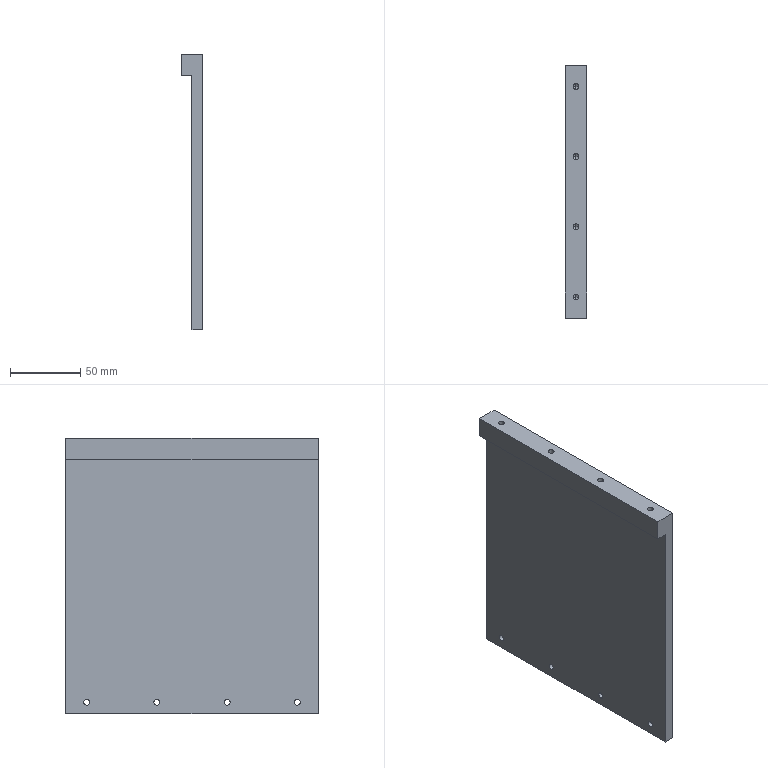Component | SolidWorks | P-SLJ-001-005-1 | 1 solid | 32 faces | box 15 x 180 x 196 mm | volume 283635 mm3 | cylinder 16 | cone 8 | plane 8 | commonest cylinder face diameters 4.2 x16 | material 45#
STEP:
#1=CARTESIAN_POINT('',(-14.213,3.346,40.769));
#2=VERTEX_POINT('',#1);
#3=CARTESIAN_POINT('',(-14.213,3.346,40.934));
#4=VERTEX_POINT('',#3);
#5=CARTESIAN_POINT('',(-14.213,3.346,40.852));
#6=DIRECTION('',(-1.,0.,0.));
#7=DIRECTION('',(0.,0.,1.));
#8=AXIS2_PLACEMENT_3D('',#5,#6,#7);
#9=CIRCLE('',#8,0.08268);
#10=EDGE_CURVE('',#2,#4,#9,.T.);
#11=ORIENTED_EDGE('',*,*,#10,.F.);
#12=CARTESIAN_POINT('',(-14.508,3.346,40.769));
#13=VERTEX_POINT('',#12);
#14=CARTESIAN_POINT('',(-14.508,3.346,40.769));
#15=DIRECTION('',(-1.,0.,0.));
#16=VECTOR('',#15,39.37);
#17=LINE('',#14,#16);
#18=EDGE_CURVE('',#2,#13,#17,.T.);
#19=ORIENTED_EDGE('',*,*,#18,.T.);
#20=CARTESIAN_POINT('',(-14.508,3.346,40.934));
#21=VERTEX_POINT('',#20);
#22=CARTESIAN_POINT('',(-14.508,3.346,40.852));
#23=DIRECTION('',(-1.,0.,0.));
#24=DIRECTION('',(0.,0.,1.));
#25=AXIS2_PLACEMENT_3D('',#22,#23,#24);
#26=CIRCLE('',#25,0.08268);
#27=EDGE_CURVE('',#13,#21,#26,.T.);
#28=ORIENTED_EDGE('',*,*,#27,.T.);
#29=CARTESIAN_POINT('',(-14.508,3.346,40.934));
#30=DIRECTION('',(-1.,0.,0.));
#31=VECTOR('',#30,39.37);
#32=LINE('',#29,#31);
#33=EDGE_CURVE('',#4,#21,#32,.T.);
#34=ORIENTED_EDGE('',*,*,#33,.F.);
#35=EDGE_LOOP('',(#11,#19,#28,#34));
#36=FACE_OUTER_BOUND('',#35,.T.);
#37=CARTESIAN_POINT('',(-14.508,3.346,40.852));
#38=DIRECTION('',(-1.,0.,0.));
#39=DIRECTION('',(0.,0.,1.));
#40=AXIS2_PLACEMENT_3D('',#37,#38,#39);
#41=CYLINDRICAL_SURFACE('',#40,0.08268);
#42=ADVANCED_FACE('',(#36),#41,.F.);
#43=CARTESIAN_POINT('',(-14.213,1.378,40.769));
#44=VERTEX_POINT('',#43);
#45=CARTESIAN_POINT('',(-14.213,1.378,40.934));
#46=VERTEX_POINT('',#45);
#47=CARTESIAN_POINT('',(-14.213,1.378,40.852));
#48=DIRECTION('',(-1.,0.,0.));
#49=DIRECTION('',(0.,0.,1.));
#50=AXIS2_PLACEMENT_3D('',#47,#48,#49);
#51=CIRCLE('',#50,0.08268);
#52=EDGE_CURVE('',#44,#46,#51,.T.);
#53=ORIENTED_EDGE('',*,*,#52,.F.);
#54=CARTESIAN_POINT('',(-14.508,1.378,40.769));
#55=VERTEX_POINT('',#54);
#56=CARTESIAN_POINT('',(-14.508,1.378,40.769));
#57=DIRECTION('',(-1.,0.,0.));
#58=VECTOR('',#57,39.37);
#59=LINE('',#56,#58);
#60=EDGE_CURVE('',#44,#55,#59,.T.);
#61=ORIENTED_EDGE('',*,*,#60,.T.);
#62=CARTESIAN_POINT('',(-14.508,1.378,40.934));
#63=VERTEX_POINT('',#62);
#64=CARTESIAN_POINT('',(-14.508,1.378,40.852));
#65=DIRECTION('',(-1.,0.,0.));
#66=DIRECTION('',(0.,0.,1.));
#67=AXIS2_PLACEMENT_3D('',#64,#65,#66);
#68=CIRCLE('',#67,0.08268);
#69=EDGE_CURVE('',#55,#63,#68,.T.);
#70=ORIENTED_EDGE('',*,*,#69,.T.);
#71=CARTESIAN_POINT('',(-14.508,1.378,40.934));
#72=DIRECTION('',(-1.,0.,0.));
#73=VECTOR('',#72,39.37);
#74=LINE('',#71,#73);
#75=EDGE_CURVE('',#46,#63,#74,.T.);
#76=ORIENTED_EDGE('',*,*,#75,.F.);
#77=EDGE_LOOP('',(#53,#61,#70,#76));
#78=FACE_OUTER_BOUND('',#77,.T.);
#79=CARTESIAN_POINT('',(-14.508,1.378,40.852));
#80=DIRECTION('',(-1.,0.,0.));
#81=DIRECTION('',(0.,0.,1.));
#82=AXIS2_PLACEMENT_3D('',#79,#80,#81);
#83=CYLINDRICAL_SURFACE('',#82,0.08268);
#84=ADVANCED_FACE('',(#78),#83,.F.);
#85=CARTESIAN_POINT('',(-14.213,-0.5906,40.769));
#86=VERTEX_POINT('',#85);
#87=CARTESIAN_POINT('',(-14.213,-0.5906,40.934));
#88=VERTEX_POINT('',#87);
#89=CARTESIAN_POINT('',(-14.213,-0.5906,40.852));
#90=DIRECTION('',(-1.,0.,0.));
#91=DIRECTION('',(0.,0.,1.));
#92=AXIS2_PLACEMENT_3D('',#89,#90,#91);
#93=CIRCLE('',#92,0.08268);
#94=EDGE_CURVE('',#86,#88,#93,.T.);
#95=ORIENTED_EDGE('',*,*,#94,.F.);
#96=CARTESIAN_POINT('',(-14.508,-0.5906,40.769));
#97=VERTEX_POINT('',#96);
#98=CARTESIAN_POINT('',(-14.508,-0.5906,40.769));
#99=DIRECTION('',(-1.,0.,0.));
#100=VECTOR('',#99,39.37);
#101=LINE('',#98,#100);
#102=EDGE_CURVE('',#86,#97,#101,.T.);
#103=ORIENTED_EDGE('',*,*,#102,.T.);
#104=CARTESIAN_POINT('',(-14.508,-0.5906,40.934));
#105=VERTEX_POINT('',#104);
#106=CARTESIAN_POINT('',(-14.508,-0.5906,40.852));
#107=DIRECTION('',(-1.,0.,0.));
#108=DIRECTION('',(0.,0.,1.));
#109=AXIS2_PLACEMENT_3D('',#106,#107,#108);
#110=CIRCLE('',#109,0.08268);
#111=EDGE_CURVE('',#97,#105,#110,.T.);
#112=ORIENTED_EDGE('',*,*,#111,.T.);
#113=CARTESIAN_POINT('',(-14.508,-0.5906,40.934));
#114=DIRECTION('',(-1.,0.,0.));
#115=VECTOR('',#114,39.37);
#116=LINE('',#113,#115);
#117=EDGE_CURVE('',#88,#105,#116,.T.);
#118=ORIENTED_EDGE('',*,*,#117,.F.);
#119=EDGE_LOOP('',(#95,#103,#112,#118));
#120=FACE_OUTER_BOUND('',#119,.T.);
#121=CARTESIAN_POINT('',(-14.508,-0.5906,40.852));
#122=DIRECTION('',(-1.,0.,0.));
#123=DIRECTION('',(0.,0.,1.));
#124=AXIS2_PLACEMENT_3D('',#121,#122,#123);
#125=CYLINDRICAL_SURFACE('',#124,0.08268);
#126=ADVANCED_FACE('',(#120),#125,.F.);
#127=CARTESIAN_POINT('',(-14.213,-2.559,40.769));
#128=VERTEX_POINT('',#127);
#129=CARTESIAN_POINT('',(-14.213,-2.559,40.934));
#130=VERTEX_POINT('',#129);
#131=CARTESIAN_POINT('',(-14.213,-2.559,40.852));
#132=DIRECTION('',(-1.,0.,0.));
#133=DIRECTION('',(0.,0.,1.));
#134=AXIS2_PLACEMENT_3D('',#131,#132,#133);
#135=CIRCLE('',#134,0.08268);
#136=EDGE_CURVE('',#128,#130,#135,.T.);
#137=ORIENTED_EDGE('',*,*,#136,.F.);
#138=CARTESIAN_POINT('',(-14.508,-2.559,40.769));
#139=VERTEX_POINT('',#138);
#140=CARTESIAN_POINT('',(-14.508,-2.559,40.769));
#141=DIRECTION('',(-1.,0.,0.));
#142=VECTOR('',#141,39.37);
#143=LINE('',#140,#142);
#144=EDGE_CURVE('',#128,#139,#143,.T.);
#145=ORIENTED_EDGE('',*,*,#144,.T.);
#146=CARTESIAN_POINT('',(-14.508,-2.559,40.934));
#147=VERTEX_POINT('',#146);
#148=CARTESIAN_POINT('',(-14.508,-2.559,40.852));
#149=DIRECTION('',(-1.,0.,0.));
#150=DIRECTION('',(0.,0.,1.));
#151=AXIS2_PLACEMENT_3D('',#148,#149,#150);
#152=CIRCLE('',#151,0.08268);
#153=EDGE_CURVE('',#139,#147,#152,.T.);
#154=ORIENTED_EDGE('',*,*,#153,.T.);
#155=CARTESIAN_POINT('',(-14.508,-2.559,40.934));
#156=DIRECTION('',(-1.,0.,0.));
#157=VECTOR('',#156,39.37);
#158=LINE('',#155,#157);
#159=EDGE_CURVE('',#130,#147,#158,.T.);
#160=ORIENTED_EDGE('',*,*,#159,.F.);
#161=EDGE_LOOP('',(#137,#145,#154,#160));
#162=FACE_OUTER_BOUND('',#161,.T.);
#163=CARTESIAN_POINT('',(-14.508,-2.559,40.852));
#164=DIRECTION('',(-1.,0.,0.));
#165=DIRECTION('',(0.,0.,1.));
#166=AXIS2_PLACEMENT_3D('',#163,#164,#165);
#167=CYLINDRICAL_SURFACE('',#166,0.08268);
#168=ADVANCED_FACE('',(#162),#167,.F.);
#169=CARTESIAN_POINT('',(-14.591,3.346,47.702));
#170=VERTEX_POINT('',#169);
#171=CARTESIAN_POINT('',(-14.425,3.346,47.702));
#172=VERTEX_POINT('',#171);
#173=CARTESIAN_POINT('',(-14.508,3.346,47.702));
#174=DIRECTION('',(0.,0.,1.));
#175=DIRECTION('',(1.,0.,0.));
#176=AXIS2_PLACEMENT_3D('',#173,#174,#175);
#177=CIRCLE('',#176,0.08268);
#178=EDGE_CURVE('',#170,#172,#177,.T.);
#179=ORIENTED_EDGE('',*,*,#178,.F.);
#180=CARTESIAN_POINT('',(-14.591,3.346,48.253));
#181=VERTEX_POINT('',#180);
#182=CARTESIAN_POINT('',(-14.591,3.346,48.253));
#183=DIRECTION('',(0.,0.,1.));
#184=VECTOR('',#183,39.37);
#185=LINE('',#182,#184);
#186=EDGE_CURVE('',#170,#181,#185,.T.);
#187=ORIENTED_EDGE('',*,*,#186,.T.);
#188=CARTESIAN_POINT('',(-14.425,3.346,48.253));
#189=VERTEX_POINT('',#188);
#190=CARTESIAN_POINT('',(-14.508,3.346,48.253));
#191=DIRECTION('',(0.,0.,1.));
#192=DIRECTION('',(1.,0.,0.));
#193=AXIS2_PLACEMENT_3D('',#190,#191,#192);
#194=CIRCLE('',#193,0.08268);
#195=EDGE_CURVE('',#181,#189,#194,.T.);
#196=ORIENTED_EDGE('',*,*,#195,.T.);
#197=CARTESIAN_POINT('',(-14.425,3.346,48.253));
#198=DIRECTION('',(0.,0.,1.));
#199=VECTOR('',#198,39.37);
#200=LINE('',#197,#199);
#201=EDGE_CURVE('',#172,#189,#200,.T.);
#202=ORIENTED_EDGE('',*,*,#201,.F.);
#203=EDGE_LOOP('',(#179,#187,#196,#202));
#204=FACE_OUTER_BOUND('',#203,.T.);
#205=CARTESIAN_POINT('',(-14.508,3.346,48.253));
#206=DIRECTION('',(0.,0.,1.));
#207=DIRECTION('',(1.,0.,0.));
#208=AXIS2_PLACEMENT_3D('',#205,#206,#207);
#209=CYLINDRICAL_SURFACE('',#208,0.08268);
#210=ADVANCED_FACE('',(#204),#209,.F.);
#211=CARTESIAN_POINT('',(-14.525,3.346,47.663));
#212=VERTEX_POINT('',#211);
#213=CARTESIAN_POINT('',(-14.508,3.329,47.663));
#214=VERTEX_POINT('',#213);
#215=CARTESIAN_POINT('',(-14.508,3.346,47.663));
#216=DIRECTION('',(0.,0.,1.));
#217=DIRECTION('',(1.,0.,0.));
#218=AXIS2_PLACEMENT_3D('',#215,#216,#217);
#219=CIRCLE('',#218,0.01715);
#220=EDGE_CURVE('',#212,#214,#219,.T.);
#221=ORIENTED_EDGE('',*,*,#220,.F.);
#222=CARTESIAN_POINT('',(-14.591,3.346,47.702));
#223=DIRECTION('',(-0.8572,0.,0.515));
#224=VECTOR('',#223,39.37);
#225=LINE('',#222,#224);
#226=EDGE_CURVE('',#212,#170,#225,.T.);
#227=ORIENTED_EDGE('',*,*,#226,.T.);
#228=ORIENTED_EDGE('',*,*,#178,.T.);
#229=CARTESIAN_POINT('',(-14.508,3.346,47.652));
#230=VERTEX_POINT('',#229);
#231=CARTESIAN_POINT('',(-14.425,3.346,47.702));
#232=DIRECTION('',(0.8572,0.,0.515));
#233=VECTOR('',#232,39.37);
#234=LINE('',#231,#233);
#235=EDGE_CURVE('',#230,#172,#234,.T.);
#236=ORIENTED_EDGE('',*,*,#235,.F.);
#237=CARTESIAN_POINT('',(-14.508,3.346,47.652));
#238=DIRECTION('',(-0.,0.8572,-0.515));
#239=VECTOR('',#238,39.37);
#240=LINE('',#237,#239);
#241=EDGE_CURVE('',#214,#230,#240,.T.);
#242=ORIENTED_EDGE('',*,*,#241,.F.);
#243=EDGE_LOOP('',(#221,#227,#228,#236,#242));
#244=FACE_OUTER_BOUND('',#243,.T.);
#245=CARTESIAN_POINT('',(-14.508,3.346,47.702));
#246=DIRECTION('',(0.,0.,1.));
#247=DIRECTION('',(1.,0.,0.));
#248=AXIS2_PLACEMENT_3D('',#245,#246,#247);
#249=CONICAL_SURFACE('',#248,0.08268,1.03);
#250=ADVANCED_FACE('',(#244),#249,.F.);
#251=CARTESIAN_POINT('',(-14.591,1.378,47.702));
#252=VERTEX_POINT('',#251);
#253=CARTESIAN_POINT('',(-14.425,1.378,47.702));
#254=VERTEX_POINT('',#253);
#255=CARTESIAN_POINT('',(-14.508,1.378,47.702));
#256=DIRECTION('',(0.,0.,1.));
#257=DIRECTION('',(1.,0.,0.));
#258=AXIS2_PLACEMENT_3D('',#255,#256,#257);
#259=CIRCLE('',#258,0.08268);
#260=EDGE_CURVE('',#252,#254,#259,.T.);
#261=ORIENTED_EDGE('',*,*,#260,.F.);
#262=CARTESIAN_POINT('',(-14.591,1.378,48.253));
#263=VERTEX_POINT('',#262);
#264=CARTESIAN_POINT('',(-14.591,1.378,48.253));
#265=DIRECTION('',(0.,0.,1.));
#266=VECTOR('',#265,39.37);
#267=LINE('',#264,#266);
#268=EDGE_CURVE('',#252,#263,#267,.T.);
#269=ORIENTED_EDGE('',*,*,#268,.T.);
#270=CARTESIAN_POINT('',(-14.425,1.378,48.253));
#271=VERTEX_POINT('',#270);
#272=CARTESIAN_POINT('',(-14.508,1.378,48.253));
#273=DIRECTION('',(0.,0.,1.));
#274=DIRECTION('',(1.,0.,0.));
#275=AXIS2_PLACEMENT_3D('',#272,#273,#274);
#276=CIRCLE('',#275,0.08268);
#277=EDGE_CURVE('',#263,#271,#276,.T.);
#278=ORIENTED_EDGE('',*,*,#277,.T.);
#279=CARTESIAN_POINT('',(-14.425,1.378,48.253));
#280=DIRECTION('',(0.,0.,1.));
#281=VECTOR('',#280,39.37);
#282=LINE('',#279,#281);
#283=EDGE_CURVE('',#254,#271,#282,.T.);
#284=ORIENTED_EDGE('',*,*,#283,.F.);
#285=EDGE_LOOP('',(#261,#269,#278,#284));
#286=FACE_OUTER_BOUND('',#285,.T.);
#287=CARTESIAN_POINT('',(-14.508,1.378,48.253));
#288=DIRECTION('',(0.,0.,1.));
#289=DIRECTION('',(1.,0.,0.));
#290=AXIS2_PLACEMENT_3D('',#287,#288,#289);
#291=CYLINDRICAL_SURFACE('',#290,0.08268);
#292=ADVANCED_FACE('',(#286),#291,.F.);
#293=CARTESIAN_POINT('',(-14.525,1.378,47.663));
#294=VERTEX_POINT('',#293);
#295=CARTESIAN_POINT('',(-14.508,1.361,47.663));
#296=VERTEX_POINT('',#295);
#297=CARTESIAN_POINT('',(-14.508,1.378,47.663));
#298=DIRECTION('',(0.,0.,1.));
#299=DIRECTION('',(1.,0.,0.));
#300=AXIS2_PLACEMENT_3D('',#297,#298,#299);
#301=CIRCLE('',#300,0.01715);
#302=EDGE_CURVE('',#294,#296,#301,.T.);
#303=ORIENTED_EDGE('',*,*,#302,.F.);
#304=CARTESIAN_POINT('',(-14.591,1.378,47.702));
#305=DIRECTION('',(-0.8572,0.,0.515));
#306=VECTOR('',#305,39.37);
#307=LINE('',#304,#306);
#308=EDGE_CURVE('',#294,#252,#307,.T.);
#309=ORIENTED_EDGE('',*,*,#308,.T.);
#310=ORIENTED_EDGE('',*,*,#260,.T.);
#311=CARTESIAN_POINT('',(-14.508,1.378,47.652));
#312=VERTEX_POINT('',#311);
#313=CARTESIAN_POINT('',(-14.425,1.378,47.702));
#314=DIRECTION('',(0.8572,0.,0.515));
#315=VECTOR('',#314,39.37);
#316=LINE('',#313,#315);
#317=EDGE_CURVE('',#312,#254,#316,.T.);
#318=ORIENTED_EDGE('',*,*,#317,.F.);
#319=CARTESIAN_POINT('',(-14.508,1.378,47.652));
#320=DIRECTION('',(-0.,0.8572,-0.515));
#321=VECTOR('',#320,39.37);
#322=LINE('',#319,#321);
#323=EDGE_CURVE('',#296,#312,#322,.T.);
#324=ORIENTED_EDGE('',*,*,#323,.F.);
#325=EDGE_LOOP('',(#303,#309,#310,#318,#324));
#326=FACE_OUTER_BOUND('',#325,.T.);
#327=CARTESIAN_POINT('',(-14.508,1.378,47.702));
#328=DIRECTION('',(0.,0.,1.));
#329=DIRECTION('',(1.,0.,0.));
#330=AXIS2_PLACEMENT_3D('',#327,#328,#329);
#331=CONICAL_SURFACE('',#330,0.08268,1.03);
#332=ADVANCED_FACE('',(#326),#331,.F.);
#333=CARTESIAN_POINT('',(-14.591,-0.5906,47.702));
#334=VERTEX_POINT('',#333);
#335=CARTESIAN_POINT('',(-14.425,-0.5906,47.702));
#336=VERTEX_POINT('',#335);
#337=CARTESIAN_POINT('',(-14.508,-0.5906,47.702));
#338=DIRECTION('',(0.,0.,1.));
#339=DIRECTION('',(1.,0.,0.));
#340=AXIS2_PLACEMENT_3D('',#337,#338,#339);
#341=CIRCLE('',#340,0.08268);
#342=EDGE_CURVE('',#334,#336,#341,.T.);
#343=ORIENTED_EDGE('',*,*,#342,.F.);
#344=CARTESIAN_POINT('',(-14.591,-0.5906,48.253));
#345=VERTEX_POINT('',#344);
#346=CARTESIAN_POINT('',(-14.591,-0.5906,48.253));
#347=DIRECTION('',(0.,0.,1.));
#348=VECTOR('',#347,39.37);
#349=LINE('',#346,#348);
#350=EDGE_CURVE('',#334,#345,#349,.T.);
#351=ORIENTED_EDGE('',*,*,#350,.T.);
#352=CARTESIAN_POINT('',(-14.425,-0.5906,48.253));
#353=VERTEX_POINT('',#352);
#354=CARTESIAN_POINT('',(-14.508,-0.5906,48.253));
#355=DIRECTION('',(0.,0.,1.));
#356=DIRECTION('',(1.,0.,0.));
#357=AXIS2_PLACEMENT_3D('',#354,#355,#356);
#358=CIRCLE('',#357,0.08268);
#359=EDGE_CURVE('',#345,#353,#358,.T.);
#360=ORIENTED_EDGE('',*,*,#359,.T.);
#361=CARTESIAN_POINT('',(-14.425,-0.5906,48.253));
#362=DIRECTION('',(0.,0.,1.));
#363=VECTOR('',#362,39.37);
#364=LINE('',#361,#363);
#365=EDGE_CURVE('',#336,#353,#364,.T.);
#366=ORIENTED_EDGE('',*,*,#365,.F.);
#367=EDGE_LOOP('',(#343,#351,#360,#366));
#368=FACE_OUTER_BOUND('',#367,.T.);
#369=CARTESIAN_POINT('',(-14.508,-0.5906,48.253));
#370=DIRECTION('',(0.,0.,1.));
#371=DIRECTION('',(1.,0.,0.));
#372=AXIS2_PLACEMENT_3D('',#369,#370,#371);
#373=CYLINDRICAL_SURFACE('',#372,0.08268);
#374=ADVANCED_FACE('',(#368),#373,.F.);
#375=CARTESIAN_POINT('',(-14.525,-0.5906,47.663));
#376=VERTEX_POINT('',#375);
#377=CARTESIAN_POINT('',(-14.508,-0.6077,47.663));
#378=VERTEX_POINT('',#377);
#379=CARTESIAN_POINT('',(-14.508,-0.5906,47.663));
#380=DIRECTION('',(0.,0.,1.));
#381=DIRECTION('',(1.,0.,0.));
#382=AXIS2_PLACEMENT_3D('',#379,#380,#381);
#383=CIRCLE('',#382,0.01715);
#384=EDGE_CURVE('',#376,#378,#383,.T.);
#385=ORIENTED_EDGE('',*,*,#384,.F.);
#386=CARTESIAN_POINT('',(-14.591,-0.5906,47.702));
#387=DIRECTION('',(-0.8572,0.,0.515));
#388=VECTOR('',#387,39.37);
#389=LINE('',#386,#388);
#390=EDGE_CURVE('',#376,#334,#389,.T.);
#391=ORIENTED_EDGE('',*,*,#390,.T.);
#392=ORIENTED_EDGE('',*,*,#342,.T.);
#393=CARTESIAN_POINT('',(-14.508,-0.5906,47.652));
#394=VERTEX_POINT('',#393);
#395=CARTESIAN_POINT('',(-14.425,-0.5906,47.702));
#396=DIRECTION('',(0.8572,0.,0.515));
#397=VECTOR('',#396,39.37);
#398=LINE('',#395,#397);
#399=EDGE_CURVE('',#394,#336,#398,.T.);
#400=ORIENTED_EDGE('',*,*,#399,.F.);
#401=CARTESIAN_POINT('',(-14.508,-0.5906,47.652));
#402=DIRECTION('',(-0.,0.8572,-0.515));
#403=VECTOR('',#402,39.37);
#404=LINE('',#401,#403);
#405=EDGE_CURVE('',#378,#394,#404,.T.);
#406=ORIENTED_EDGE('',*,*,#405,.F.);
#407=EDGE_LOOP('',(#385,#391,#392,#400,#406));
#408=FACE_OUTER_BOUND('',#407,.T.);
#409=CARTESIAN_POINT('',(-14.508,-0.5906,47.702));
#410=DIRECTION('',(0.,0.,1.));
#411=DIRECTION('',(1.,0.,0.));
#412=AXIS2_PLACEMENT_3D('',#409,#410,#411);
#413=CONICAL_SURFACE('',#412,0.08268,1.03);
#414=ADVANCED_FACE('',(#408),#413,.F.);
#415=CARTESIAN_POINT('',(-14.591,-2.559,47.702));
#416=VERTEX_POINT('',#415);
#417=CARTESIAN_POINT('',(-14.425,-2.559,47.702));
#418=VERTEX_POINT('',#417);
#419=CARTESIAN_POINT('',(-14.508,-2.559,47.702));
#420=DIRECTION('',(0.,0.,1.));
#421=DIRECTION('',(1.,0.,0.));
#422=AXIS2_PLACEMENT_3D('',#419,#420,#421);
#423=CIRCLE('',#422,0.08268);
#424=EDGE_CURVE('',#416,#418,#423,.T.);
#425=ORIENTED_EDGE('',*,*,#424,.F.);
#426=CARTESIAN_POINT('',(-14.591,-2.559,48.253));
#427=VERTEX_POINT('',#426);
#428=CARTESIAN_POINT('',(-14.591,-2.559,48.253));
#429=DIRECTION('',(0.,0.,1.));
#430=VECTOR('',#429,39.37);
#431=LINE('',#428,#430);
#432=EDGE_CURVE('',#416,#427,#431,.T.);
#433=ORIENTED_EDGE('',*,*,#432,.T.);
#434=CARTESIAN_POINT('',(-14.425,-2.559,48.253));
#435=VERTEX_POINT('',#434);
#436=CARTESIAN_POINT('',(-14.508,-2.559,48.253));
#437=DIRECTION('',(0.,0.,1.));
#438=DIRECTION('',(1.,0.,0.));
#439=AXIS2_PLACEMENT_3D('',#436,#437,#438);
#440=CIRCLE('',#439,0.08268);
#441=EDGE_CURVE('',#427,#435,#440,.T.);
#442=ORIENTED_EDGE('',*,*,#441,.T.);
#443=CARTESIAN_POINT('',(-14.425,-2.559,48.253));
#444=DIRECTION('',(0.,0.,1.));
#445=VECTOR('',#444,39.37);
#446=LINE('',#443,#445);
#447=EDGE_CURVE('',#418,#435,#446,.T.);
#448=ORIENTED_EDGE('',*,*,#447,.F.);
#449=EDGE_LOOP('',(#425,#433,#442,#448));
#450=FACE_OUTER_BOUND('',#449,.T.);
#451=CARTESIAN_POINT('',(-14.508,-2.559,48.253));
#452=DIRECTION('',(0.,0.,1.));
#453=DIRECTION('',(1.,0.,0.));
#454=AXIS2_PLACEMENT_3D('',#451,#452,#453);
#455=CYLINDRICAL_SURFACE('',#454,0.08268);
#456=ADVANCED_FACE('',(#450),#455,.F.);
#457=CARTESIAN_POINT('',(-14.525,-2.559,47.663));
#458=VERTEX_POINT('',#457);
#459=CARTESIAN_POINT('',(-14.508,-2.576,47.663));
#460=VERTEX_POINT('',#459);
#461=CARTESIAN_POINT('',(-14.508,-2.559,47.663));
#462=DIRECTION('',(0.,0.,1.));
#463=DIRECTION('',(1.,0.,0.));
#464=AXIS2_PLACEMENT_3D('',#461,#462,#463);
#465=CIRCLE('',#464,0.01715);
#466=EDGE_CURVE('',#458,#460,#465,.T.);
#467=ORIENTED_EDGE('',*,*,#466,.F.);
#468=CARTESIAN_POINT('',(-14.591,-2.559,47.702));
#469=DIRECTION('',(-0.8572,0.,0.515));
#470=VECTOR('',#469,39.37);
#471=LINE('',#468,#470);
#472=EDGE_CURVE('',#458,#416,#471,.T.);
#473=ORIENTED_EDGE('',*,*,#472,.T.);
#474=ORIENTED_EDGE('',*,*,#424,.T.);
#475=CARTESIAN_POINT('',(-14.508,-2.559,47.652));
#476=VERTEX_POINT('',#475);
#477=CARTESIAN_POINT('',(-14.425,-2.559,47.702));
#478=DIRECTION('',(0.8572,0.,0.515));
#479=VECTOR('',#478,39.37);
#480=LINE('',#477,#479);
#481=EDGE_CURVE('',#476,#418,#480,.T.);
#482=ORIENTED_EDGE('',*,*,#481,.F.);
#483=CARTESIAN_POINT('',(-14.508,-2.559,47.652));
#484=DIRECTION('',(-0.,0.8572,-0.515));
#485=VECTOR('',#484,39.37);
#486=LINE('',#483,#485);
#487=EDGE_CURVE('',#460,#476,#486,.T.);
#488=ORIENTED_EDGE('',*,*,#487,.F.);
#489=EDGE_LOOP('',(#467,#473,#474,#482,#488));
#490=FACE_OUTER_BOUND('',#489,.T.);
#491=CARTESIAN_POINT('',(-14.508,-2.559,47.702));
#492=DIRECTION('',(0.,0.,1.));
#493=DIRECTION('',(1.,0.,0.));
#494=AXIS2_PLACEMENT_3D('',#491,#492,#493);
#495=CONICAL_SURFACE('',#494,0.08268,1.03);
#496=ADVANCED_FACE('',(#490),#495,.F.);
#497=CARTESIAN_POINT('',(-14.508,3.346,48.253));
#498=DIRECTION('',(0.,0.,1.));
#499=DIRECTION('',(1.,0.,0.));
#500=AXIS2_PLACEMENT_3D('',#497,#498,#499);
#501=CIRCLE('',#500,0.08268);
#502=EDGE_CURVE('',#189,#181,#501,.T.);
#503=ORIENTED_EDGE('',*,*,#502,.F.);
#504=ORIENTED_EDGE('',*,*,#195,.F.);
#505=EDGE_LOOP('',(#503,#504));
#506=FACE_BOUND('',#505,.T.);
#507=CARTESIAN_POINT('',(-14.508,1.378,48.253));
#508=DIRECTION('',(0.,0.,1.));
#509=DIRECTION('',(1.,0.,0.));
#510=AXIS2_PLACEMENT_3D('',#507,#508,#509);
#511=CIRCLE('',#510,0.08268);
#512=EDGE_CURVE('',#271,#263,#511,.T.);
#513=ORIENTED_EDGE('',*,*,#512,.F.);
#514=ORIENTED_EDGE('',*,*,#277,.F.);
#515=EDGE_LOOP('',(#513,#514));
#516=FACE_BOUND('',#515,.T.);
#517=CARTESIAN_POINT('',(-14.508,-0.5906,48.253));
#518=DIRECTION('',(0.,0.,1.));
#519=DIRECTION('',(1.,0.,0.));
#520=AXIS2_PLACEMENT_3D('',#517,#518,#519);
#521=CIRCLE('',#520,0.08268);
#522=EDGE_CURVE('',#353,#345,#521,.T.);
#523=ORIENTED_EDGE('',*,*,#522,.F.);
#524=ORIENTED_EDGE('',*,*,#359,.F.);
#525=EDGE_LOOP('',(#523,#524));
#526=FACE_BOUND('',#525,.T.);
#527=CARTESIAN_POINT('',(-14.508,-2.559,48.253));
#528=DIRECTION('',(0.,0.,1.));
#529=DIRECTION('',(1.,0.,0.));
#530=AXIS2_PLACEMENT_3D('',#527,#528,#529);
#531=CIRCLE('',#530,0.08268);
#532=EDGE_CURVE('',#435,#427,#531,.T.);
#533=ORIENTED_EDGE('',*,*,#532,.F.);
#534=ORIENTED_EDGE('',*,*,#441,.F.);
#535=EDGE_LOOP('',(#533,#534));
#536=FACE_BOUND('',#535,.T.);
#537=CARTESIAN_POINT('',(-14.803,-3.15,48.253));
#538=VERTEX_POINT('',#537);
#539=CARTESIAN_POINT('',(-14.213,-3.15,48.253));
#540=VERTEX_POINT('',#539);
#541=CARTESIAN_POINT('',(-14.803,-3.15,48.253));
#542=DIRECTION('',(1.,0.,0.));
#543=VECTOR('',#542,39.37);
#544=LINE('',#541,#543);
#545=EDGE_CURVE('',#538,#540,#544,.T.);
#546=ORIENTED_EDGE('',*,*,#545,.T.);
#547=CARTESIAN_POINT('',(-14.213,3.937,48.253));
#548=VERTEX_POINT('',#547);
#549=CARTESIAN_POINT('',(-14.213,3.937,48.253));
#550=DIRECTION('',(0.,-1.,0.));
#551=VECTOR('',#550,39.37);
#552=LINE('',#549,#551);
#553=EDGE_CURVE('',#548,#540,#552,.T.);
#554=ORIENTED_EDGE('',*,*,#553,.F.);
#555=CARTESIAN_POINT('',(-14.803,3.937,48.253));
#556=VERTEX_POINT('',#555);
#557=CARTESIAN_POINT('',(-14.803,3.937,48.253));
#558=DIRECTION('',(1.,0.,0.));
#559=VECTOR('',#558,39.37);
#560=LINE('',#557,#559);
#561=EDGE_CURVE('',#556,#548,#560,.T.);
#562=ORIENTED_EDGE('',*,*,#561,.F.);
#563=CARTESIAN_POINT('',(-14.803,3.937,48.253));
#564=DIRECTION('',(0.,-1.,0.));
#565=VECTOR('',#564,39.37);
#566=LINE('',#563,#565);
#567=EDGE_CURVE('',#556,#538,#566,.T.);
#568=ORIENTED_EDGE('',*,*,#567,.T.);
#569=EDGE_LOOP('',(#546,#554,#562,#568));
#570=FACE_OUTER_BOUND('',#569,.T.);
#571=CARTESIAN_POINT('',(-14.803,3.937,48.253));
#572=DIRECTION('',(0.,0.,-1.));
#573=DIRECTION('',(-1.,0.,0.));
#574=AXIS2_PLACEMENT_3D('',#571,#572,#573);
#575=PLANE('',#574);
#576=ADVANCED_FACE('',(#506,#516,#526,#536,#570),#575,.F.);
#577=CARTESIAN_POINT('',(-14.213,3.346,40.852));
#578=DIRECTION('',(-1.,0.,0.));
#579=DIRECTION('',(0.,0.,1.));
#580=AXIS2_PLACEMENT_3D('',#577,#578,#579);
#581=CIRCLE('',#580,0.08268);
#582=EDGE_CURVE('',#4,#2,#581,.T.);
#583=ORIENTED_EDGE('',*,*,#582,.T.);
#584=ORIENTED_EDGE('',*,*,#10,.T.);
#585=EDGE_LOOP('',(#583,#584));
#586=FACE_BOUND('',#585,.T.);
#587=CARTESIAN_POINT('',(-14.213,1.378,40.852));
#588=DIRECTION('',(-1.,0.,0.));
#589=DIRECTION('',(0.,0.,1.));
#590=AXIS2_PLACEMENT_3D('',#587,#588,#589);
#591=CIRCLE('',#590,0.08268);
#592=EDGE_CURVE('',#46,#44,#591,.T.);
#593=ORIENTED_EDGE('',*,*,#592,.T.);
#594=ORIENTED_EDGE('',*,*,#52,.T.);
#595=EDGE_LOOP('',(#593,#594));
#596=FACE_BOUND('',#595,.T.);
#597=CARTESIAN_POINT('',(-14.213,-0.5906,40.852));
#598=DIRECTION('',(-1.,0.,0.));
#599=DIRECTION('',(0.,0.,1.));
#600=AXIS2_PLACEMENT_3D('',#597,#598,#599);
#601=CIRCLE('',#600,0.08268);
#602=EDGE_CURVE('',#88,#86,#601,.T.);
#603=ORIENTED_EDGE('',*,*,#602,.T.);
#604=ORIENTED_EDGE('',*,*,#94,.T.);
#605=EDGE_LOOP('',(#603,#604));
#606=FACE_BOUND('',#605,.T.);
#607=CARTESIAN_POINT('',(-14.213,-2.559,40.852));
#608=DIRECTION('',(-1.,0.,0.));
#609=DIRECTION('',(0.,0.,1.));
#610=AXIS2_PLACEMENT_3D('',#607,#608,#609);
#611=CIRCLE('',#610,0.08268);
#612=EDGE_CURVE('',#130,#128,#611,.T.);
#613=ORIENTED_EDGE('',*,*,#612,.T.);
#614=ORIENTED_EDGE('',*,*,#136,.T.);
#615=EDGE_LOOP('',(#613,#614));
#616=FACE_BOUND('',#615,.T.);
#617=CARTESIAN_POINT('',(-14.213,-3.15,40.537));
#618=VERTEX_POINT('',#617);
#619=CARTESIAN_POINT('',(-14.213,-3.15,48.253));
#620=DIRECTION('',(-0.,0.,-1.));
#621=VECTOR('',#620,39.37);
#622=LINE('',#619,#621);
#623=EDGE_CURVE('',#540,#618,#622,.T.);
#624=ORIENTED_EDGE('',*,*,#623,.T.);
#625=CARTESIAN_POINT('',(-14.213,3.937,40.537));
#626=VERTEX_POINT('',#625);
#627=CARTESIAN_POINT('',(-14.213,3.937,40.537));
#628=DIRECTION('',(0.,-1.,0.));
#629=VECTOR('',#628,39.37);
#630=LINE('',#627,#629);
#631=EDGE_CURVE('',#626,#618,#630,.T.);
#632=ORIENTED_EDGE('',*,*,#631,.F.);
#633=CARTESIAN_POINT('',(-14.213,3.937,48.253));
#634=DIRECTION('',(-0.,0.,-1.));
#635=VECTOR('',#634,39.37);
#636=LINE('',#633,#635);
#637=EDGE_CURVE('',#548,#626,#636,.T.);
#638=ORIENTED_EDGE('',*,*,#637,.F.);
#639=ORIENTED_EDGE('',*,*,#553,.T.);
#640=EDGE_LOOP('',(#624,#632,#638,#639));
#641=FACE_OUTER_BOUND('',#640,.T.);
#642=CARTESIAN_POINT('',(-14.213,3.937,48.253));
#643=DIRECTION('',(-1.,0.,0.));
#644=DIRECTION('',(0.,0.,1.));
#645=AXIS2_PLACEMENT_3D('',#642,#643,#644);
#646=PLANE('',#645);
#647=ADVANCED_FACE('',(#586,#596,#606,#616,#641),#646,.F.);
#648=CARTESIAN_POINT('',(-14.508,-3.15,40.537));
#649=VERTEX_POINT('',#648);
#650=CARTESIAN_POINT('',(-14.508,-3.15,40.537));
#651=DIRECTION('',(-1.,0.,0.));
#652=VECTOR('',#651,39.37);
#653=LINE('',#650,#652);
#654=EDGE_CURVE('',#618,#649,#653,.T.);
#655=ORIENTED_EDGE('',*,*,#654,.T.);
#656=CARTESIAN_POINT('',(-14.508,3.937,40.537));
#657=VERTEX_POINT('',#656);
#658=CARTESIAN_POINT('',(-14.508,3.937,40.537));
#659=DIRECTION('',(0.,-1.,0.));
#660=VECTOR('',#659,39.37);
#661=LINE('',#658,#660);
#662=EDGE_CURVE('',#657,#649,#661,.T.);
#663=ORIENTED_EDGE('',*,*,#662,.F.);
#664=CARTESIAN_POINT('',(-14.508,3.937,40.537));
#665=DIRECTION('',(-1.,0.,0.));
#666=VECTOR('',#665,39.37);
#667=LINE('',#664,#666);
#668=EDGE_CURVE('',#626,#657,#667,.T.);
#669=ORIENTED_EDGE('',*,*,#668,.F.);
#670=ORIENTED_EDGE('',*,*,#631,.T.);
#671=EDGE_LOOP('',(#655,#663,#669,#670));
#672=FACE_OUTER_BOUND('',#671,.T.);
#673=CARTESIAN_POINT('',(-14.508,3.937,40.537));
#674=DIRECTION('',(0.,0.,1.));
#675=DIRECTION('',(1.,0.,0.));
#676=AXIS2_PLACEMENT_3D('',#673,#674,#675);
#677=PLANE('',#676);
#678=ADVANCED_FACE('',(#672),#677,.F.);
#679=CARTESIAN_POINT('',(-14.508,3.346,40.852));
#680=DIRECTION('',(-1.,0.,0.));
#681=DIRECTION('',(0.,0.,1.));
#682=AXIS2_PLACEMENT_3D('',#679,#680,#681);
#683=CIRCLE('',#682,0.08268);
#684=EDGE_CURVE('',#21,#13,#683,.T.);
#685=ORIENTED_EDGE('',*,*,#684,.F.);
#686=ORIENTED_EDGE('',*,*,#27,.F.);
#687=EDGE_LOOP('',(#685,#686));
#688=FACE_BOUND('',#687,.T.);
#689=CARTESIAN_POINT('',(-14.508,1.378,40.852));
#690=DIRECTION('',(-1.,0.,0.));
#691=DIRECTION('',(0.,0.,1.));
#692=AXIS2_PLACEMENT_3D('',#689,#690,#691);
#693=CIRCLE('',#692,0.08268);
#694=EDGE_CURVE('',#63,#55,#693,.T.);
#695=ORIENTED_EDGE('',*,*,#694,.F.);
#696=ORIENTED_EDGE('',*,*,#69,.F.);
#697=EDGE_LOOP('',(#695,#696));
#698=FACE_BOUND('',#697,.T.);
#699=CARTESIAN_POINT('',(-14.508,-0.5906,40.852));
#700=DIRECTION('',(-1.,0.,0.));
#701=DIRECTION('',(0.,0.,1.));
#702=AXIS2_PLACEMENT_3D('',#699,#700,#701);
#703=CIRCLE('',#702,0.08268);
#704=EDGE_CURVE('',#105,#97,#703,.T.);
#705=ORIENTED_EDGE('',*,*,#704,.F.);
#706=ORIENTED_EDGE('',*,*,#111,.F.);
#707=EDGE_LOOP('',(#705,#706));
#708=FACE_BOUND('',#707,.T.);
#709=CARTESIAN_POINT('',(-14.508,-2.559,40.852));
#710=DIRECTION('',(-1.,0.,0.));
#711=DIRECTION('',(0.,0.,1.));
#712=AXIS2_PLACEMENT_3D('',#709,#710,#711);
#713=CIRCLE('',#712,0.08268);
#714=EDGE_CURVE('',#147,#139,#713,.T.);
#715=ORIENTED_EDGE('',*,*,#714,.F.);
#716=ORIENTED_EDGE('',*,*,#153,.F.);
#717=EDGE_LOOP('',(#715,#716));
#718=FACE_BOUND('',#717,.T.);
#719=ORIENTED_EDGE('',*,*,#241,.T.);
#720=CARTESIAN_POINT('',(-14.508,3.364,47.663));
#721=VERTEX_POINT('',#720);
#722=CARTESIAN_POINT('',(-14.508,3.346,47.652));
#723=DIRECTION('',(0.,0.8572,0.515));
#724=VECTOR('',#723,39.37);
#725=LINE('',#722,#724);
#726=EDGE_CURVE('',#230,#721,#725,.T.);
#727=ORIENTED_EDGE('',*,*,#726,.T.);
#728=CARTESIAN_POINT('',(-14.508,3.937,47.663));
#729=VERTEX_POINT('',#728);
#730=CARTESIAN_POINT('',(-14.508,3.937,47.663));
#731=DIRECTION('',(0.,-1.,0.));
#732=VECTOR('',#731,39.37);
#733=LINE('',#730,#732);
#734=EDGE_CURVE('',#729,#721,#733,.T.);
#735=ORIENTED_EDGE('',*,*,#734,.F.);
#736=CARTESIAN_POINT('',(-14.508,3.937,40.537));
#737=DIRECTION('',(0.,0.,1.));
#738=VECTOR('',#737,39.37);
#739=LINE('',#736,#738);
#740=EDGE_CURVE('',#657,#729,#739,.T.);
#741=ORIENTED_EDGE('',*,*,#740,.F.);
#742=ORIENTED_EDGE('',*,*,#662,.T.);
#743=CARTESIAN_POINT('',(-14.508,-3.15,47.663));
#744=VERTEX_POINT('',#743);
#745=CARTESIAN_POINT('',(-14.508,-3.15,40.537));
#746=DIRECTION('',(0.,0.,1.));
#747=VECTOR('',#746,39.37);
#748=LINE('',#745,#747);
#749=EDGE_CURVE('',#649,#744,#748,.T.);
#750=ORIENTED_EDGE('',*,*,#749,.T.);
#751=CARTESIAN_POINT('',(-14.508,3.937,47.663));
#752=DIRECTION('',(0.,-1.,0.));
#753=VECTOR('',#752,39.37);
#754=LINE('',#751,#753);
#755=EDGE_CURVE('',#460,#744,#754,.T.);
#756=ORIENTED_EDGE('',*,*,#755,.F.);
#757=ORIENTED_EDGE('',*,*,#487,.T.);
#758=CARTESIAN_POINT('',(-14.508,-2.542,47.663));
#759=VERTEX_POINT('',#758);
#760=CARTESIAN_POINT('',(-14.508,-2.559,47.652));
#761=DIRECTION('',(0.,0.8572,0.515));
#762=VECTOR('',#761,39.37);
#763=LINE('',#760,#762);
#764=EDGE_CURVE('',#476,#759,#763,.T.);
#765=ORIENTED_EDGE('',*,*,#764,.T.);
#766=CARTESIAN_POINT('',(-14.508,3.937,47.663));
#767=DIRECTION('',(0.,-1.,0.));
#768=VECTOR('',#767,39.37);
#769=LINE('',#766,#768);
#770=EDGE_CURVE('',#378,#759,#769,.T.);
#771=ORIENTED_EDGE('',*,*,#770,.F.);
#772=ORIENTED_EDGE('',*,*,#405,.T.);
#773=CARTESIAN_POINT('',(-14.508,-0.5734,47.663));
#774=VERTEX_POINT('',#773);
#775=CARTESIAN_POINT('',(-14.508,-0.5906,47.652));
#776=DIRECTION('',(0.,0.8572,0.515));
#777=VECTOR('',#776,39.37);
#778=LINE('',#775,#777);
#779=EDGE_CURVE('',#394,#774,#778,.T.);
#780=ORIENTED_EDGE('',*,*,#779,.T.);
#781=CARTESIAN_POINT('',(-14.508,3.937,47.663));
#782=DIRECTION('',(0.,-1.,0.));
#783=VECTOR('',#782,39.37);
#784=LINE('',#781,#783);
#785=EDGE_CURVE('',#296,#774,#784,.T.);
#786=ORIENTED_EDGE('',*,*,#785,.F.);
#787=ORIENTED_EDGE('',*,*,#323,.T.);
#788=CARTESIAN_POINT('',(-14.508,1.395,47.663));
#789=VERTEX_POINT('',#788);
#790=CARTESIAN_POINT('',(-14.508,1.378,47.652));
#791=DIRECTION('',(0.,0.8572,0.515));
#792=VECTOR('',#791,39.37);
#793=LINE('',#790,#792);
#794=EDGE_CURVE('',#312,#789,#793,.T.);
#795=ORIENTED_EDGE('',*,*,#794,.T.);
#796=CARTESIAN_POINT('',(-14.508,3.937,47.663));
#797=DIRECTION('',(0.,-1.,0.));
#798=VECTOR('',#797,39.37);
#799=LINE('',#796,#798);
#800=EDGE_CURVE('',#214,#789,#799,.T.);
#801=ORIENTED_EDGE('',*,*,#800,.F.);
#802=EDGE_LOOP('',(#719,#727,#735,#741,#742,#750,#756,#757,#765,#771,#772,#780,#786,#787,#795,#801));
#803=FACE_OUTER_BOUND('',#802,.T.);
#804=CARTESIAN_POINT('',(-14.508,3.937,40.537));
#805=DIRECTION('',(1.,0.,-0.));
#806=DIRECTION('',(-0.,0.,-1.));
#807=AXIS2_PLACEMENT_3D('',#804,#805,#806);
#808=PLANE('',#807);
#809=ADVANCED_FACE('',(#688,#698,#708,#718,#803),#808,.F.);
#810=ORIENTED_EDGE('',*,*,#734,.T.);
#811=CARTESIAN_POINT('',(-14.508,3.346,47.663));
#812=DIRECTION('',(0.,0.,1.));
#813=DIRECTION('',(1.,0.,0.));
#814=AXIS2_PLACEMENT_3D('',#811,#812,#813);
#815=CIRCLE('',#814,0.01715);
#816=EDGE_CURVE('',#721,#212,#815,.T.);
#817=ORIENTED_EDGE('',*,*,#816,.T.);
#818=ORIENTED_EDGE('',*,*,#220,.T.);
#819=ORIENTED_EDGE('',*,*,#800,.T.);
#820=CARTESIAN_POINT('',(-14.508,1.378,47.663));
#821=DIRECTION('',(0.,0.,1.));
#822=DIRECTION('',(1.,0.,0.));
#823=AXIS2_PLACEMENT_3D('',#820,#821,#822);
#824=CIRCLE('',#823,0.01715);
#825=EDGE_CURVE('',#789,#294,#824,.T.);
#826=ORIENTED_EDGE('',*,*,#825,.T.);
#827=ORIENTED_EDGE('',*,*,#302,.T.);
#828=ORIENTED_EDGE('',*,*,#785,.T.);
#829=CARTESIAN_POINT('',(-14.508,-0.5906,47.663));
#830=DIRECTION('',(0.,0.,1.));
#831=DIRECTION('',(1.,0.,0.));
#832=AXIS2_PLACEMENT_3D('',#829,#830,#831);
#833=CIRCLE('',#832,0.01715);
#834=EDGE_CURVE('',#774,#376,#833,.T.);
#835=ORIENTED_EDGE('',*,*,#834,.T.);
#836=ORIENTED_EDGE('',*,*,#384,.T.);
#837=ORIENTED_EDGE('',*,*,#770,.T.);
#838=CARTESIAN_POINT('',(-14.508,-2.559,47.663));
#839=DIRECTION('',(0.,0.,1.));
#840=DIRECTION('',(1.,0.,0.));
#841=AXIS2_PLACEMENT_3D('',#838,#839,#840);
#842=CIRCLE('',#841,0.01715);
#843=EDGE_CURVE('',#759,#458,#842,.T.);
#844=ORIENTED_EDGE('',*,*,#843,.T.);
#845=ORIENTED_EDGE('',*,*,#466,.T.);
#846=ORIENTED_EDGE('',*,*,#755,.T.);
#847=CARTESIAN_POINT('',(-14.803,-3.15,47.663));
#848=VERTEX_POINT('',#847);
#849=CARTESIAN_POINT('',(-14.803,-3.15,47.663));
#850=DIRECTION('',(-1.,0.,0.));
#851=VECTOR('',#850,39.37);
#852=LINE('',#849,#851);
#853=EDGE_CURVE('',#744,#848,#852,.T.);
#854=ORIENTED_EDGE('',*,*,#853,.T.);
#855=CARTESIAN_POINT('',(-14.803,3.937,47.663));
#856=VERTEX_POINT('',#855);
#857=CARTESIAN_POINT('',(-14.803,3.937,47.663));
#858=DIRECTION('',(0.,-1.,0.));
#859=VECTOR('',#858,39.37);
#860=LINE('',#857,#859);
#861=EDGE_CURVE('',#856,#848,#860,.T.);
#862=ORIENTED_EDGE('',*,*,#861,.F.);
#863=CARTESIAN_POINT('',(-14.803,3.937,47.663));
#864=DIRECTION('',(-1.,0.,0.));
#865=VECTOR('',#864,39.37);
#866=LINE('',#863,#865);
#867=EDGE_CURVE('',#729,#856,#866,.T.);
#868=ORIENTED_EDGE('',*,*,#867,.F.);
#869=EDGE_LOOP('',(#810,#817,#818,#819,#826,#827,#828,#835,#836,#837,#844,#845,#846,#854,#862,#868));
#870=FACE_OUTER_BOUND('',#869,.T.);
#871=CARTESIAN_POINT('',(-14.803,3.937,47.663));
#872=DIRECTION('',(0.,0.,1.));
#873=DIRECTION('',(1.,0.,0.));
#874=AXIS2_PLACEMENT_3D('',#871,#872,#873);
#875=PLANE('',#874);
#876=ADVANCED_FACE('',(#870),#875,.F.);
#877=CARTESIAN_POINT('',(-14.803,-3.15,48.253));
#878=DIRECTION('',(0.,0.,1.));
#879=VECTOR('',#878,39.37);
#880=LINE('',#877,#879);
#881=EDGE_CURVE('',#848,#538,#880,.T.);
#882=ORIENTED_EDGE('',*,*,#881,.T.);
#883=ORIENTED_EDGE('',*,*,#567,.F.);
#884=CARTESIAN_POINT('',(-14.803,3.937,48.253));
#885=DIRECTION('',(0.,0.,1.));
#886=VECTOR('',#885,39.37);
#887=LINE('',#884,#886);
#888=EDGE_CURVE('',#856,#556,#887,.T.);
#889=ORIENTED_EDGE('',*,*,#888,.F.);
#890=ORIENTED_EDGE('',*,*,#861,.T.);
#891=EDGE_LOOP('',(#882,#883,#889,#890));
#892=FACE_OUTER_BOUND('',#891,.T.);
#893=CARTESIAN_POINT('',(-14.803,3.937,48.253));
#894=DIRECTION('',(1.,0.,-0.));
#895=DIRECTION('',(-0.,0.,-1.));
#896=AXIS2_PLACEMENT_3D('',#893,#894,#895);
#897=PLANE('',#896);
#898=ADVANCED_FACE('',(#892),#897,.F.);
#899=ORIENTED_EDGE('',*,*,#561,.T.);
#900=ORIENTED_EDGE('',*,*,#637,.T.);
#901=ORIENTED_EDGE('',*,*,#668,.T.);
#902=ORIENTED_EDGE('',*,*,#740,.T.);
#903=ORIENTED_EDGE('',*,*,#867,.T.);
#904=ORIENTED_EDGE('',*,*,#888,.T.);
#905=EDGE_LOOP('',(#899,#900,#901,#902,#903,#904));
#906=FACE_OUTER_BOUND('',#905,.T.);
#907=CARTESIAN_POINT('',(-14.803,3.937,48.253));
#908=DIRECTION('',(0.,1.,0.));
#909=DIRECTION('',(-1.,0.,0.));
#910=AXIS2_PLACEMENT_3D('',#907,#908,#909);
#911=PLANE('',#910);
#912=ADVANCED_FACE('',(#906),#911,.T.);
#913=ORIENTED_EDGE('',*,*,#545,.F.);
#914=ORIENTED_EDGE('',*,*,#881,.F.);
#915=ORIENTED_EDGE('',*,*,#853,.F.);
#916=ORIENTED_EDGE('',*,*,#749,.F.);
#917=ORIENTED_EDGE('',*,*,#654,.F.);
#918=ORIENTED_EDGE('',*,*,#623,.F.);
#919=EDGE_LOOP('',(#913,#914,#915,#916,#917,#918));
#920=FACE_OUTER_BOUND('',#919,.T.);
#921=CARTESIAN_POINT('',(-14.803,-3.15,48.253));
#922=DIRECTION('',(0.,1.,0.));
#923=DIRECTION('',(-1.,0.,0.));
#924=AXIS2_PLACEMENT_3D('',#921,#922,#923);
#925=PLANE('',#924);
#926=ADVANCED_FACE('',(#920),#925,.F.);
#927=ORIENTED_EDGE('',*,*,#472,.F.);
#928=ORIENTED_EDGE('',*,*,#843,.F.);
#929=ORIENTED_EDGE('',*,*,#764,.F.);
#930=ORIENTED_EDGE('',*,*,#481,.T.);
#931=CARTESIAN_POINT('',(-14.508,-2.559,47.702));
#932=DIRECTION('',(0.,0.,1.));
#933=DIRECTION('',(1.,0.,0.));
#934=AXIS2_PLACEMENT_3D('',#931,#932,#933);
#935=CIRCLE('',#934,0.08268);
#936=EDGE_CURVE('',#418,#416,#935,.T.);
#937=ORIENTED_EDGE('',*,*,#936,.T.);
#938=EDGE_LOOP('',(#927,#928,#929,#930,#937));
#939=FACE_OUTER_BOUND('',#938,.T.);
#940=CARTESIAN_POINT('',(-14.508,-2.559,47.702));
#941=DIRECTION('',(0.,0.,1.));
#942=DIRECTION('',(1.,0.,0.));
#943=AXIS2_PLACEMENT_3D('',#940,#941,#942);
#944=CONICAL_SURFACE('',#943,0.08268,1.03);
#945=ADVANCED_FACE('',(#939),#944,.F.);
#946=ORIENTED_EDGE('',*,*,#432,.F.);
#947=ORIENTED_EDGE('',*,*,#936,.F.);
#948=ORIENTED_EDGE('',*,*,#447,.T.);
#949=ORIENTED_EDGE('',*,*,#532,.T.);
#950=EDGE_LOOP('',(#946,#947,#948,#949));
#951=FACE_OUTER_BOUND('',#950,.T.);
#952=CARTESIAN_POINT('',(-14.508,-2.559,48.253));
#953=DIRECTION('',(0.,0.,1.));
#954=DIRECTION('',(1.,0.,0.));
#955=AXIS2_PLACEMENT_3D('',#952,#953,#954);
#956=CYLINDRICAL_SURFACE('',#955,0.08268);
#957=ADVANCED_FACE('',(#951),#956,.F.);
#958=ORIENTED_EDGE('',*,*,#390,.F.);
#959=ORIENTED_EDGE('',*,*,#834,.F.);
#960=ORIENTED_EDGE('',*,*,#779,.F.);
#961=ORIENTED_EDGE('',*,*,#399,.T.);
#962=CARTESIAN_POINT('',(-14.508,-0.5906,47.702));
#963=DIRECTION('',(0.,0.,1.));
#964=DIRECTION('',(1.,0.,0.));
#965=AXIS2_PLACEMENT_3D('',#962,#963,#964);
#966=CIRCLE('',#965,0.08268);
#967=EDGE_CURVE('',#336,#334,#966,.T.);
#968=ORIENTED_EDGE('',*,*,#967,.T.);
#969=EDGE_LOOP('',(#958,#959,#960,#961,#968));
#970=FACE_OUTER_BOUND('',#969,.T.);
#971=CARTESIAN_POINT('',(-14.508,-0.5906,47.702));
#972=DIRECTION('',(0.,0.,1.));
#973=DIRECTION('',(1.,0.,0.));
#974=AXIS2_PLACEMENT_3D('',#971,#972,#973);
#975=CONICAL_SURFACE('',#974,0.08268,1.03);
#976=ADVANCED_FACE('',(#970),#975,.F.);
#977=ORIENTED_EDGE('',*,*,#350,.F.);
#978=ORIENTED_EDGE('',*,*,#967,.F.);
#979=ORIENTED_EDGE('',*,*,#365,.T.);
#980=ORIENTED_EDGE('',*,*,#522,.T.);
#981=EDGE_LOOP('',(#977,#978,#979,#980));
#982=FACE_OUTER_BOUND('',#981,.T.);
#983=CARTESIAN_POINT('',(-14.508,-0.5906,48.253));
#984=DIRECTION('',(0.,0.,1.));
#985=DIRECTION('',(1.,0.,0.));
#986=AXIS2_PLACEMENT_3D('',#983,#984,#985);
#987=CYLINDRICAL_SURFACE('',#986,0.08268);
#988=ADVANCED_FACE('',(#982),#987,.F.);
#989=ORIENTED_EDGE('',*,*,#308,.F.);
#990=ORIENTED_EDGE('',*,*,#825,.F.);
#991=ORIENTED_EDGE('',*,*,#794,.F.);
#992=ORIENTED_EDGE('',*,*,#317,.T.);
#993=CARTESIAN_POINT('',(-14.508,1.378,47.702));
#994=DIRECTION('',(0.,0.,1.));
#995=DIRECTION('',(1.,0.,0.));
#996=AXIS2_PLACEMENT_3D('',#993,#994,#995);
#997=CIRCLE('',#996,0.08268);
#998=EDGE_CURVE('',#254,#252,#997,.T.);
#999=ORIENTED_EDGE('',*,*,#998,.T.);
#1000=EDGE_LOOP('',(#989,#990,#991,#992,#999));
#1001=FACE_OUTER_BOUND('',#1000,.T.);
#1002=CARTESIAN_POINT('',(-14.508,1.378,47.702));
#1003=DIRECTION('',(0.,0.,1.));
#1004=DIRECTION('',(1.,0.,0.));
#1005=AXIS2_PLACEMENT_3D('',#1002,#1003,#1004);
#1006=CONICAL_SURFACE('',#1005,0.08268,1.03);
#1007=ADVANCED_FACE('',(#1001),#1006,.F.);
#1008=ORIENTED_EDGE('',*,*,#268,.F.);
#1009=ORIENTED_EDGE('',*,*,#998,.F.);
#1010=ORIENTED_EDGE('',*,*,#283,.T.);
#1011=ORIENTED_EDGE('',*,*,#512,.T.);
#1012=EDGE_LOOP('',(#1008,#1009,#1010,#1011));
#1013=FACE_OUTER_BOUND('',#1012,.T.);
#1014=CARTESIAN_POINT('',(-14.508,1.378,48.253));
#1015=DIRECTION('',(0.,0.,1.));
#1016=DIRECTION('',(1.,0.,0.));
#1017=AXIS2_PLACEMENT_3D('',#1014,#1015,#1016);
#1018=CYLINDRICAL_SURFACE('',#1017,0.08268);
#1019=ADVANCED_FACE('',(#1013),#1018,.F.);
#1020=ORIENTED_EDGE('',*,*,#226,.F.);
#1021=ORIENTED_EDGE('',*,*,#816,.F.);
#1022=ORIENTED_EDGE('',*,*,#726,.F.);
#1023=ORIENTED_EDGE('',*,*,#235,.T.);
#1024=CARTESIAN_POINT('',(-14.508,3.346,47.702));
#1025=DIRECTION('',(0.,0.,1.));
#1026=DIRECTION('',(1.,0.,0.));
#1027=AXIS2_PLACEMENT_3D('',#1024,#1025,#1026);
#1028=CIRCLE('',#1027,0.08268);
#1029=EDGE_CURVE('',#172,#170,#1028,.T.);
#1030=ORIENTED_EDGE('',*,*,#1029,.T.);
#1031=EDGE_LOOP('',(#1020,#1021,#1022,#1023,#1030));
#1032=FACE_OUTER_BOUND('',#1031,.T.);
#1033=CARTESIAN_POINT('',(-14.508,3.346,47.702));
#1034=DIRECTION('',(0.,0.,1.));
#1035=DIRECTION('',(1.,0.,0.));
#1036=AXIS2_PLACEMENT_3D('',#1033,#1034,#1035);
#1037=CONICAL_SURFACE('',#1036,0.08268,1.03);
#1038=ADVANCED_FACE('',(#1032),#1037,.F.);
#1039=ORIENTED_EDGE('',*,*,#186,.F.);
#1040=ORIENTED_EDGE('',*,*,#1029,.F.);
#1041=ORIENTED_EDGE('',*,*,#201,.T.);
#1042=ORIENTED_EDGE('',*,*,#502,.T.);
#1043=EDGE_LOOP('',(#1039,#1040,#1041,#1042));
#1044=FACE_OUTER_BOUND('',#1043,.T.);
#1045=CARTESIAN_POINT('',(-14.508,3.346,48.253));
#1046=DIRECTION('',(0.,0.,1.));
#1047=DIRECTION('',(1.,0.,0.));
#1048=AXIS2_PLACEMENT_3D('',#1045,#1046,#1047);
#1049=CYLINDRICAL_SURFACE('',#1048,0.08268);
#1050=ADVANCED_FACE('',(#1044),#1049,.F.);
#1051=ORIENTED_EDGE('',*,*,#144,.F.);
#1052=ORIENTED_EDGE('',*,*,#612,.F.);
#1053=ORIENTED_EDGE('',*,*,#159,.T.);
#1054=ORIENTED_EDGE('',*,*,#714,.T.);
#1055=EDGE_LOOP('',(#1051,#1052,#1053,#1054));
#1056=FACE_OUTER_BOUND('',#1055,.T.);
#1057=CARTESIAN_POINT('',(-14.508,-2.559,40.852));
#1058=DIRECTION('',(-1.,0.,0.));
#1059=DIRECTION('',(0.,0.,1.));
#1060=AXIS2_PLACEMENT_3D('',#1057,#1058,#1059);
#1061=CYLINDRICAL_SURFACE('',#1060,0.08268);
#1062=ADVANCED_FACE('',(#1056),#1061,.F.);
#1063=ORIENTED_EDGE('',*,*,#102,.F.);
#1064=ORIENTED_EDGE('',*,*,#602,.F.);
#1065=ORIENTED_EDGE('',*,*,#117,.T.);
#1066=ORIENTED_EDGE('',*,*,#704,.T.);
#1067=EDGE_LOOP('',(#1063,#1064,#1065,#1066));
#1068=FACE_OUTER_BOUND('',#1067,.T.);
#1069=CARTESIAN_POINT('',(-14.508,-0.5906,40.852));
#1070=DIRECTION('',(-1.,0.,0.));
#1071=DIRECTION('',(0.,0.,1.));
#1072=AXIS2_PLACEMENT_3D('',#1069,#1070,#1071);
#1073=CYLINDRICAL_SURFACE('',#1072,0.08268);
#1074=ADVANCED_FACE('',(#1068),#1073,.F.);
#1075=ORIENTED_EDGE('',*,*,#60,.F.);
#1076=ORIENTED_EDGE('',*,*,#592,.F.);
#1077=ORIENTED_EDGE('',*,*,#75,.T.);
#1078=ORIENTED_EDGE('',*,*,#694,.T.);
#1079=EDGE_LOOP('',(#1075,#1076,#1077,#1078));
#1080=FACE_OUTER_BOUND('',#1079,.T.);
#1081=CARTESIAN_POINT('',(-14.508,1.378,40.852));
#1082=DIRECTION('',(-1.,0.,0.));
#1083=DIRECTION('',(0.,0.,1.));
#1084=AXIS2_PLACEMENT_3D('',#1081,#1082,#1083);
#1085=CYLINDRICAL_SURFACE('',#1084,0.08268);
#1086=ADVANCED_FACE('',(#1080),#1085,.F.);
#1087=ORIENTED_EDGE('',*,*,#18,.F.);
#1088=ORIENTED_EDGE('',*,*,#582,.F.);
#1089=ORIENTED_EDGE('',*,*,#33,.T.);
#1090=ORIENTED_EDGE('',*,*,#684,.T.);
#1091=EDGE_LOOP('',(#1087,#1088,#1089,#1090));
#1092=FACE_OUTER_BOUND('',#1091,.T.);
#1093=CARTESIAN_POINT('',(-14.508,3.346,40.852));
#1094=DIRECTION('',(-1.,0.,0.));
#1095=DIRECTION('',(0.,0.,1.));
#1096=AXIS2_PLACEMENT_3D('',#1093,#1094,#1095);
#1097=CYLINDRICAL_SURFACE('',#1096,0.08268);
#1098=ADVANCED_FACE('',(#1092),#1097,.F.);
#1099=CLOSED_SHELL('',(#42,#84,#126,#168,#210,#250,#292,#332,#374,#414,#456,#496,#576,#647,#678,#809,#876,#898,#912,#926,#945,#957,#976,#988,#1007,#1019,#1038,#1050,#1062,#1074,#1086,#1098));
#1100=MANIFOLD_SOLID_BREP('',#1099);
#1101=CARTESIAN_POINT('',(0.,0.,0.));
#1102=DIRECTION('',(0.,0.,1.));
#1103=DIRECTION('',(1.,0.,0.));
#1104=AXIS2_PLACEMENT_3D('',#1101,#1102,#1103);
#1105=(LENGTH_UNIT()NAMED_UNIT(*)SI_UNIT($,.METRE.));
#1106=LENGTH_MEASURE_WITH_UNIT(LENGTH_MEASURE(0.0254),#1105);
#1107=DIMENSIONAL_EXPONENTS(1.,0.,0.,0.,0.,0.,0.);
#1108=(CONVERSION_BASED_UNIT('',#1106)LENGTH_UNIT()NAMED_UNIT(#1107));
#1109=UNCERTAINTY_MEASURE_WITH_UNIT(LENGTH_MEASURE(0.00001),#1108,'','');
#1110=(NAMED_UNIT(*)PLANE_ANGLE_UNIT()SI_UNIT($,.RADIAN.));
#1111=(NAMED_UNIT(*)SI_UNIT($,.STERADIAN.)SOLID_ANGLE_UNIT());
#1112=(GEOMETRIC_REPRESENTATION_CONTEXT(3)GLOBAL_UNCERTAINTY_ASSIGNED_CONTEXT((#1109))GLOBAL_UNIT_ASSIGNED_CONTEXT((#1108,#1110,#1111))REPRESENTATION_CONTEXT('',''));
#1113=ADVANCED_BREP_SHAPE_REPRESENTATION('',(#1100,#1104),#1112);
#1114=COLOUR_RGB('',0.7922,0.8196,0.9333);
#1115=FILL_AREA_STYLE_COLOUR('',#1114);
#1116=FILL_AREA_STYLE('',(#1115));
#1117=SURFACE_STYLE_FILL_AREA(#1116);
#1118=SURFACE_SIDE_STYLE('',(#1117));
#1119=SURFACE_STYLE_USAGE(.BOTH.,#1118);
#1120=PRESENTATION_STYLE_ASSIGNMENT((#1119));
#1121=STYLED_ITEM('',(#1120),#1100);
#1122=PRESENTATION_LAYER_ASSIGNMENT('','',(#1121));
#1123=(LENGTH_UNIT()NAMED_UNIT(*)SI_UNIT($,.METRE.));
#1124=LENGTH_MEASURE_WITH_UNIT(LENGTH_MEASURE(0.0254),#1123);
#1125=DIMENSIONAL_EXPONENTS(1.,0.,0.,0.,0.,0.,0.);
#1126=(CONVERSION_BASED_UNIT('',#1124)LENGTH_UNIT()NAMED_UNIT(#1125));
#1127=UNCERTAINTY_MEASURE_WITH_UNIT(LENGTH_MEASURE(0.00001),#1126,'','');
#1128=(NAMED_UNIT(*)PLANE_ANGLE_UNIT()SI_UNIT($,.RADIAN.));
#1129=(NAMED_UNIT(*)SI_UNIT($,.STERADIAN.)SOLID_ANGLE_UNIT());
#1130=(GEOMETRIC_REPRESENTATION_CONTEXT(3)GLOBAL_UNCERTAINTY_ASSIGNED_CONTEXT((#1127))GLOBAL_UNIT_ASSIGNED_CONTEXT((#1126,#1128,#1129))REPRESENTATION_CONTEXT('',''));
#1131=MECHANICAL_DESIGN_GEOMETRIC_PRESENTATION_REPRESENTATION('',(#1121),#1130);